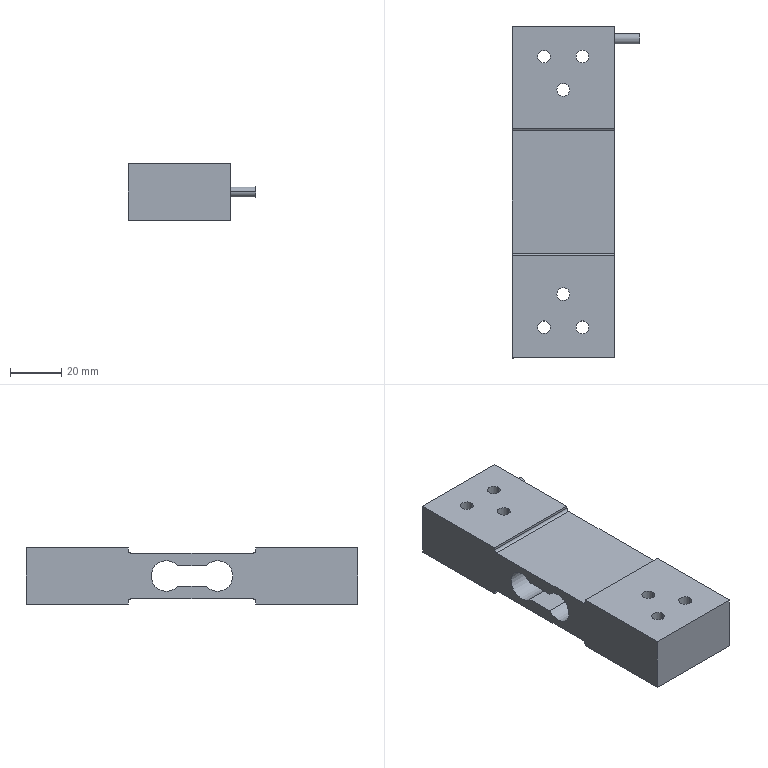Component | SolidWorks | WeightSensor100KgNew-1 | 1 solid | 38 faces | box 50 x 130 x 22 mm | volume 92053 mm3 | cylinder 21 | plane 17 | commonest cylinder face diameters 5 x12 2 x4 12 x3 4 x2
build123d program:
from build123d import *

# Parameters (mm, degrees)
SKETCH1_W           = 130
SKETCH1_H           = 40
BOSS_EXTRUDE1_DEPTH = 22
SKETCH2_W           = 50
SKETCH2_H           = 4
CUT_EXTRUDE1_DEPTH  = 47
FILLET1_R           = 1
SKETCH3_R           = 2
CUT_EXTRUDE2_DEPTH  = 47
M6_TAPPED_HOLE1_D   = 5
SKETCH7_R           = 2
BOSS_EXTRUDE2_DEPTH = 10


with BuildPart() as part:
    # Sketch1 → Boss-Extrude1 (new body)
    with BuildSketch(Plane(origin=(0, 0, 0), x_dir=(1, 0, 0), z_dir=(0, 1, 0))):
        Rectangle(SKETCH1_W, SKETCH1_H)
    extrude(amount=BOSS_EXTRUDE1_DEPTH)

    # Sketch2 → Cut-Extrude1 (cut)
    with BuildSketch(Plane.XY.offset(20)):
        with Locations((0, 22)):
            Rectangle(SKETCH2_W, SKETCH2_H)
        Rectangle(SKETCH2_W, SKETCH2_H)
        with BuildLine():
            Line((-5.528, 7), (5.528, 7))
            ThreePointArc((5.528, 7), (16, 11), (5.528, 15))
            Line((5.528, 15), (-5.528, 15))
            ThreePointArc((-5.528, 15), (-16, 11), (-5.528, 7))
        make_face()
    extrude(amount=-CUT_EXTRUDE1_DEPTH, mode=Mode.SUBTRACT)

    # Fillet1
    fillet1_edges = [part.edges().sort_by_distance(p)[0] for p in [
        (25, 20, 0),
        (-25, 20, 0),
        (-25, 2, 0),
        (25, 2, 0),
    ]]
    fillet(fillet1_edges, radius=FILLET1_R)

    # Sketch3 → Cut-Extrude2 (cut)
    with BuildSketch(Plane(origin=(0, 22, 0), x_dir=(1, 0, 0), z_dir=(0, 1, 0))):
        with Locations(Location((-40, 0, 0), (0, 0, 270))):
            Circle(SKETCH3_R)
        with Locations(Location((-53, 7.5, 0), (0, 0, 270))):
            Circle(SKETCH3_R)
        with Locations(Location((-53, -7.5, 0), (0, 0, 270))):
            Circle(SKETCH3_R)
        with Locations(Location((40, 0, 0), (0, 0, 270))):
            Circle(SKETCH3_R)
        with Locations(Location((53, 7.5, 0), (0, 0, 270))):
            Circle(SKETCH3_R)
        with Locations(Location((53, -7.5, 0), (0, 0, 270))):
            Circle(SKETCH3_R)
    extrude(amount=-CUT_EXTRUDE2_DEPTH, mode=Mode.SUBTRACT)

    # M6 Tapped Hole1 (through all)
    with Locations(Plane(origin=(0, 22, 0), x_dir=(1, 0, 0), z_dir=(0, 1, 0))):
        with Locations((-53, 7.5), (-40, 0), (-53, -7.5), (40, 0), (53, 7.5), (53, -7.5)):
            Hole(M6_TAPPED_HOLE1_D / 2)

    # Sketch7 → Boss-Extrude2 (add)
    with BuildSketch(Plane.XY.offset(20)):
        with Locations(Location((-60, 11, 0), (0, 0, 180))):
            Circle(SKETCH7_R)
    extrude(amount=BOSS_EXTRUDE2_DEPTH)


solid = part.part

# Placed as in the assembly
solid = solid.moved(Location((1140.186, 1093.312, 1428.454), (-90, 90, 0)))